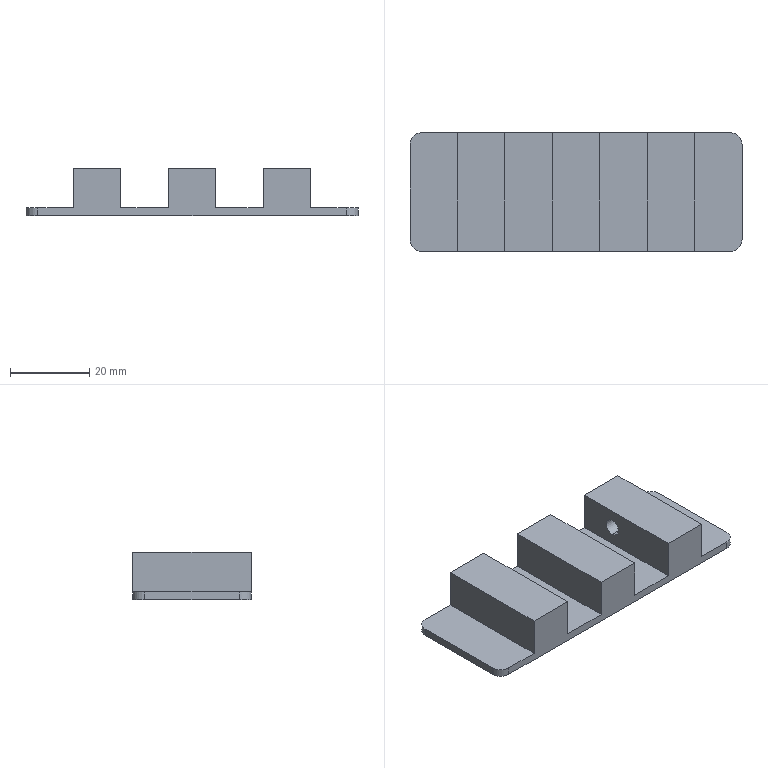Component | SolidWorks | SecondGenerationFour-sidedLabelingFeedingAdjustmentBaffle-1 | 1 solid | 24 faces | box 84 x 30 x 12 mm | volume 15658 mm3 | plane 18 | cylinder 6 | commonest cylinder face diameters 6 x4 4.2 x2
build123d program:
from build123d import *

# Parameters (mm, degrees)
SKETCH1_W             = 84
SKETCH1_H             = 30
BOSS_EXTRUDE1_DEPTH   = 6
SKETCH2_W             = 20
SKETCH2_H             = 53.944
SKETCH2_W_2           = 12
SKETCH2_H_2           = 79.849
SKETCH2_W_3           = 22.276
SKETCH2_H_3           = 76.76
CUT_EXTRUDE1_DEPTH    = 10
M5_TAPPED_HOLE1_D     = 4.2
M5_TAPPED_HOLE1_DEPTH = 19
M5_TAPPED_HOLE1_TIP   = 1.262
FILLET1_R             = 3


with BuildPart() as part:
    # Sketch1 → Boss-Extrude1 (new, symmetric)
    with BuildSketch(Plane.XY):
        Rectangle(SKETCH1_W, SKETCH1_H)
    extrude(amount=BOSS_EXTRUDE1_DEPTH, both=True)

    # Sketch2 → Cut-Extrude1 (cut)
    with BuildSketch(Plane.XY.offset(6)):
        with Locations((40, -0.6636)):
            Rectangle(SKETCH2_W, SKETCH2_H)
        with Locations((12, -0.6636)):
            Rectangle(SKETCH2_W_2, SKETCH2_H)
        with Locations((-12, 2.902)):
            Rectangle(SKETCH2_W_2, SKETCH2_H_2)
        with Locations((-41.138, 15.701)):
            Rectangle(SKETCH2_W_3, SKETCH2_H_3)
    extrude(amount=-CUT_EXTRUDE1_DEPTH, mode=Mode.SUBTRACT)

    # M5 Tapped Hole1
    with Locations(Plane(origin=(30, 0, 0), x_dir=(0, 0, -1), z_dir=(1, 0, 0))):
        with Locations((-1, 5)):
            Hole(M5_TAPPED_HOLE1_D / 2, depth=M5_TAPPED_HOLE1_DEPTH)
            with Locations((0, 0, -(M5_TAPPED_HOLE1_DEPTH + M5_TAPPED_HOLE1_TIP / 2))):  # 118° drill point
                Cone(0, M5_TAPPED_HOLE1_D / 2, M5_TAPPED_HOLE1_TIP, mode=Mode.SUBTRACT)

    # Fillet1
    fillet1_edges = [part.edges().sort_by_distance(p)[0] for p in [
        (42, -15, -5),
        (42, 15, -5),
        (-42, -15, -5),
        (-42, 15, -5),
    ]]
    fillet(fillet1_edges, radius=FILLET1_R)


solid = part.part

# Placed as in the assembly
solid = solid.moved(Location((9.973, 64.131, -120), (0, 0, 0)))
STEP:
#1=CARTESIAN_POINT('',(1.101,2.722,-4.602));
#2=VERTEX_POINT('',#1);
#3=CARTESIAN_POINT('',(1.101,2.722,-4.768));
#4=VERTEX_POINT('',#3);
#5=CARTESIAN_POINT('',(1.101,2.722,-4.685));
#6=DIRECTION('',(1.,0.,0.));
#7=DIRECTION('',(0.,1.,0.));
#8=AXIS2_PLACEMENT_3D('',#5,#6,#7);
#9=CIRCLE('',#8,0.08268);
#10=EDGE_CURVE('',#2,#4,#9,.T.);
#11=ORIENTED_EDGE('',*,*,#10,.F.);
#12=CARTESIAN_POINT('',(1.574,2.722,-4.602));
#13=VERTEX_POINT('',#12);
#14=CARTESIAN_POINT('',(1.574,2.722,-4.602));
#15=DIRECTION('',(1.,0.,0.));
#16=VECTOR('',#15,39.37);
#17=LINE('',#14,#16);
#18=EDGE_CURVE('',#2,#13,#17,.T.);
#19=ORIENTED_EDGE('',*,*,#18,.T.);
#20=CARTESIAN_POINT('',(1.574,2.722,-4.768));
#21=VERTEX_POINT('',#20);
#22=CARTESIAN_POINT('',(1.574,2.722,-4.685));
#23=DIRECTION('',(1.,0.,0.));
#24=DIRECTION('',(0.,0.,-1.));
#25=AXIS2_PLACEMENT_3D('',#22,#23,#24);
#26=CIRCLE('',#25,0.08268);
#27=EDGE_CURVE('',#13,#21,#26,.T.);
#28=ORIENTED_EDGE('',*,*,#27,.T.);
#29=CARTESIAN_POINT('',(1.574,2.722,-4.768));
#30=DIRECTION('',(1.,0.,0.));
#31=VECTOR('',#30,39.37);
#32=LINE('',#29,#31);
#33=EDGE_CURVE('',#4,#21,#32,.T.);
#34=ORIENTED_EDGE('',*,*,#33,.F.);
#35=EDGE_LOOP('',(#11,#19,#28,#34));
#36=FACE_OUTER_BOUND('',#35,.T.);
#37=CARTESIAN_POINT('',(1.574,2.722,-4.685));
#38=DIRECTION('',(1.,0.,0.));
#39=DIRECTION('',(0.,0.,-1.));
#40=AXIS2_PLACEMENT_3D('',#37,#38,#39);
#41=CYLINDRICAL_SURFACE('',#40,0.08268);
#42=ADVANCED_FACE('',(#36),#41,.F.);
#43=CARTESIAN_POINT('',(-1.261,2.997,-4.961));
#44=VERTEX_POINT('',#43);
#45=CARTESIAN_POINT('',(-1.261,2.052,-4.961));
#46=VERTEX_POINT('',#45);
#47=CARTESIAN_POINT('',(-1.261,1.934,-4.961));
#48=DIRECTION('',(0.,-1.,0.));
#49=VECTOR('',#48,39.37);
#50=LINE('',#47,#49);
#51=EDGE_CURVE('',#44,#46,#50,.T.);
#52=ORIENTED_EDGE('',*,*,#51,.T.);
#53=CARTESIAN_POINT('',(-1.261,2.052,-4.882));
#54=VERTEX_POINT('',#53);
#55=CARTESIAN_POINT('',(-1.261,2.052,-4.488));
#56=DIRECTION('',(0.,0.,1.));
#57=VECTOR('',#56,39.37);
#58=LINE('',#55,#57);
#59=EDGE_CURVE('',#46,#54,#58,.T.);
#60=ORIENTED_EDGE('',*,*,#59,.T.);
#61=CARTESIAN_POINT('',(-1.261,2.997,-4.882));
#62=VERTEX_POINT('',#61);
#63=CARTESIAN_POINT('',(-1.261,1.934,-4.882));
#64=DIRECTION('',(0.,-1.,0.));
#65=VECTOR('',#64,39.37);
#66=LINE('',#63,#65);
#67=EDGE_CURVE('',#62,#54,#66,.T.);
#68=ORIENTED_EDGE('',*,*,#67,.F.);
#69=CARTESIAN_POINT('',(-1.261,2.997,-4.488));
#70=DIRECTION('',(0.,0.,-1.));
#71=VECTOR('',#70,39.37);
#72=LINE('',#69,#71);
#73=EDGE_CURVE('',#62,#44,#72,.T.);
#74=ORIENTED_EDGE('',*,*,#73,.T.);
#75=EDGE_LOOP('',(#52,#60,#68,#74));
#76=FACE_OUTER_BOUND('',#75,.T.);
#77=CARTESIAN_POINT('',(-1.261,1.934,-4.488));
#78=DIRECTION('',(1.,0.,0.));
#79=DIRECTION('',(0.,0.,-1.));
#80=AXIS2_PLACEMENT_3D('',#77,#78,#79);
#81=PLANE('',#80);
#82=ADVANCED_FACE('',(#76),#81,.F.);
#83=CARTESIAN_POINT('',(-0.316,3.115,-4.488));
#84=VERTEX_POINT('',#83);
#85=CARTESIAN_POINT('',(-0.7885,3.115,-4.488));
#86=VERTEX_POINT('',#85);
#87=CARTESIAN_POINT('',(-1.261,3.115,-4.488));
#88=DIRECTION('',(-1.,0.,0.));
#89=VECTOR('',#88,39.37);
#90=LINE('',#87,#89);
#91=EDGE_CURVE('',#84,#86,#90,.T.);
#92=ORIENTED_EDGE('',*,*,#91,.T.);
#93=CARTESIAN_POINT('',(-0.7885,1.934,-4.488));
#94=VERTEX_POINT('',#93);
#95=CARTESIAN_POINT('',(-0.7885,4.654,-4.488));
#96=DIRECTION('',(-0.,1.,0.));
#97=VECTOR('',#96,39.37);
#98=LINE('',#95,#97);
#99=EDGE_CURVE('',#94,#86,#98,.T.);
#100=ORIENTED_EDGE('',*,*,#99,.F.);
#101=CARTESIAN_POINT('',(-0.316,1.934,-4.488));
#102=VERTEX_POINT('',#101);
#103=CARTESIAN_POINT('',(-1.261,1.934,-4.488));
#104=DIRECTION('',(1.,0.,0.));
#105=VECTOR('',#104,39.37);
#106=LINE('',#103,#105);
#107=EDGE_CURVE('',#94,#102,#106,.T.);
#108=ORIENTED_EDGE('',*,*,#107,.T.);
#109=CARTESIAN_POINT('',(-0.316,4.211,-4.488));
#110=DIRECTION('',(0.,-1.,0.));
#111=VECTOR('',#110,39.37);
#112=LINE('',#109,#111);
#113=EDGE_CURVE('',#84,#102,#112,.T.);
#114=ORIENTED_EDGE('',*,*,#113,.F.);
#115=EDGE_LOOP('',(#92,#100,#108,#114));
#116=FACE_OUTER_BOUND('',#115,.T.);
#117=CARTESIAN_POINT('',(2.046,3.115,-4.488));
#118=DIRECTION('',(0.,0.,-1.));
#119=DIRECTION('',(-1.,0.,0.));
#120=AXIS2_PLACEMENT_3D('',#117,#118,#119);
#121=PLANE('',#120);
#122=ADVANCED_FACE('',(#116),#121,.F.);
#123=CARTESIAN_POINT('',(0.6289,3.115,-4.488));
#124=VERTEX_POINT('',#123);
#125=CARTESIAN_POINT('',(0.1564,3.115,-4.488));
#126=VERTEX_POINT('',#125);
#127=CARTESIAN_POINT('',(-1.261,3.115,-4.488));
#128=DIRECTION('',(-1.,0.,0.));
#129=VECTOR('',#128,39.37);
#130=LINE('',#127,#129);
#131=EDGE_CURVE('',#124,#126,#130,.T.);
#132=ORIENTED_EDGE('',*,*,#131,.T.);
#133=CARTESIAN_POINT('',(0.1564,1.934,-4.488));
#134=VERTEX_POINT('',#133);
#135=CARTESIAN_POINT('',(0.1564,4.211,-4.488));
#136=DIRECTION('',(-0.,1.,0.));
#137=VECTOR('',#136,39.37);
#138=LINE('',#135,#137);
#139=EDGE_CURVE('',#134,#126,#138,.T.);
#140=ORIENTED_EDGE('',*,*,#139,.F.);
#141=CARTESIAN_POINT('',(0.6289,1.934,-4.488));
#142=VERTEX_POINT('',#141);
#143=CARTESIAN_POINT('',(-1.261,1.934,-4.488));
#144=DIRECTION('',(1.,0.,0.));
#145=VECTOR('',#144,39.37);
#146=LINE('',#143,#145);
#147=EDGE_CURVE('',#134,#142,#146,.T.);
#148=ORIENTED_EDGE('',*,*,#147,.T.);
#149=CARTESIAN_POINT('',(0.6289,3.115,-4.488));
#150=DIRECTION('',(-0.,1.,0.));
#151=VECTOR('',#150,39.37);
#152=LINE('',#149,#151);
#153=EDGE_CURVE('',#142,#124,#152,.T.);
#154=ORIENTED_EDGE('',*,*,#153,.T.);
#155=EDGE_LOOP('',(#132,#140,#148,#154));
#156=FACE_OUTER_BOUND('',#155,.T.);
#157=CARTESIAN_POINT('',(2.046,3.115,-4.488));
#158=DIRECTION('',(0.,0.,-1.));
#159=DIRECTION('',(-1.,0.,0.));
#160=AXIS2_PLACEMENT_3D('',#157,#158,#159);
#161=PLANE('',#160);
#162=ADVANCED_FACE('',(#156),#161,.F.);
#163=CARTESIAN_POINT('',(2.046,2.052,-4.882));
#164=VERTEX_POINT('',#163);
#165=CARTESIAN_POINT('',(2.046,2.997,-4.882));
#166=VERTEX_POINT('',#165);
#167=CARTESIAN_POINT('',(2.046,1.934,-4.882));
#168=DIRECTION('',(0.,1.,0.));
#169=VECTOR('',#168,39.37);
#170=LINE('',#167,#169);
#171=EDGE_CURVE('',#164,#166,#170,.T.);
#172=ORIENTED_EDGE('',*,*,#171,.F.);
#173=CARTESIAN_POINT('',(2.046,2.052,-4.961));
#174=VERTEX_POINT('',#173);
#175=CARTESIAN_POINT('',(2.046,2.052,-4.488));
#176=DIRECTION('',(0.,0.,-1.));
#177=VECTOR('',#176,39.37);
#178=LINE('',#175,#177);
#179=EDGE_CURVE('',#164,#174,#178,.T.);
#180=ORIENTED_EDGE('',*,*,#179,.T.);
#181=CARTESIAN_POINT('',(2.046,2.997,-4.961));
#182=VERTEX_POINT('',#181);
#183=CARTESIAN_POINT('',(2.046,1.934,-4.961));
#184=DIRECTION('',(0.,1.,0.));
#185=VECTOR('',#184,39.37);
#186=LINE('',#183,#185);
#187=EDGE_CURVE('',#174,#182,#186,.T.);
#188=ORIENTED_EDGE('',*,*,#187,.T.);
#189=CARTESIAN_POINT('',(2.046,2.997,-4.488));
#190=DIRECTION('',(0.,0.,1.));
#191=VECTOR('',#190,39.37);
#192=LINE('',#189,#191);
#193=EDGE_CURVE('',#182,#166,#192,.T.);
#194=ORIENTED_EDGE('',*,*,#193,.T.);
#195=EDGE_LOOP('',(#172,#180,#188,#194));
#196=FACE_OUTER_BOUND('',#195,.T.);
#197=CARTESIAN_POINT('',(2.046,1.934,-4.488));
#198=DIRECTION('',(-1.,0.,0.));
#199=DIRECTION('',(0.,0.,1.));
#200=AXIS2_PLACEMENT_3D('',#197,#198,#199);
#201=PLANE('',#200);
#202=ADVANCED_FACE('',(#196),#201,.F.);
#203=CARTESIAN_POINT('',(1.928,3.115,-4.961));
#204=VERTEX_POINT('',#203);
#205=CARTESIAN_POINT('',(-1.143,3.115,-4.961));
#206=VERTEX_POINT('',#205);
#207=CARTESIAN_POINT('',(-1.261,3.115,-4.961));
#208=DIRECTION('',(-1.,0.,0.));
#209=VECTOR('',#208,39.37);
#210=LINE('',#207,#209);
#211=EDGE_CURVE('',#204,#206,#210,.T.);
#212=ORIENTED_EDGE('',*,*,#211,.T.);
#213=CARTESIAN_POINT('',(-1.143,3.115,-4.882));
#214=VERTEX_POINT('',#213);
#215=CARTESIAN_POINT('',(-1.143,3.115,-4.488));
#216=DIRECTION('',(0.,0.,1.));
#217=VECTOR('',#216,39.37);
#218=LINE('',#215,#217);
#219=EDGE_CURVE('',#206,#214,#218,.T.);
#220=ORIENTED_EDGE('',*,*,#219,.T.);
#221=CARTESIAN_POINT('',(-0.7885,3.115,-4.882));
#222=VERTEX_POINT('',#221);
#223=CARTESIAN_POINT('',(-1.261,3.115,-4.882));
#224=DIRECTION('',(-1.,0.,0.));
#225=VECTOR('',#224,39.37);
#226=LINE('',#223,#225);
#227=EDGE_CURVE('',#222,#214,#226,.T.);
#228=ORIENTED_EDGE('',*,*,#227,.F.);
#229=CARTESIAN_POINT('',(-0.7885,3.115,-4.488));
#230=DIRECTION('',(0.,0.,1.));
#231=VECTOR('',#230,39.37);
#232=LINE('',#229,#231);
#233=EDGE_CURVE('',#222,#86,#232,.T.);
#234=ORIENTED_EDGE('',*,*,#233,.T.);
#235=ORIENTED_EDGE('',*,*,#91,.F.);
#236=CARTESIAN_POINT('',(-0.316,3.115,-4.882));
#237=VERTEX_POINT('',#236);
#238=CARTESIAN_POINT('',(-0.316,3.115,-4.488));
#239=DIRECTION('',(0.,0.,-1.));
#240=VECTOR('',#239,39.37);
#241=LINE('',#238,#240);
#242=EDGE_CURVE('',#84,#237,#241,.T.);
#243=ORIENTED_EDGE('',*,*,#242,.T.);
#244=CARTESIAN_POINT('',(0.1564,3.115,-4.882));
#245=VERTEX_POINT('',#244);
#246=CARTESIAN_POINT('',(-1.261,3.115,-4.882));
#247=DIRECTION('',(-1.,0.,0.));
#248=VECTOR('',#247,39.37);
#249=LINE('',#246,#248);
#250=EDGE_CURVE('',#245,#237,#249,.T.);
#251=ORIENTED_EDGE('',*,*,#250,.F.);
#252=CARTESIAN_POINT('',(0.1564,3.115,-4.488));
#253=DIRECTION('',(0.,0.,1.));
#254=VECTOR('',#253,39.37);
#255=LINE('',#252,#254);
#256=EDGE_CURVE('',#245,#126,#255,.T.);
#257=ORIENTED_EDGE('',*,*,#256,.T.);
#258=ORIENTED_EDGE('',*,*,#131,.F.);
#259=CARTESIAN_POINT('',(0.6289,3.115,-4.882));
#260=VERTEX_POINT('',#259);
#261=CARTESIAN_POINT('',(0.6289,3.115,-4.488));
#262=DIRECTION('',(0.,0.,-1.));
#263=VECTOR('',#262,39.37);
#264=LINE('',#261,#263);
#265=EDGE_CURVE('',#124,#260,#264,.T.);
#266=ORIENTED_EDGE('',*,*,#265,.T.);
#267=CARTESIAN_POINT('',(1.101,3.115,-4.882));
#268=VERTEX_POINT('',#267);
#269=CARTESIAN_POINT('',(-1.261,3.115,-4.882));
#270=DIRECTION('',(-1.,0.,0.));
#271=VECTOR('',#270,39.37);
#272=LINE('',#269,#271);
#273=EDGE_CURVE('',#268,#260,#272,.T.);
#274=ORIENTED_EDGE('',*,*,#273,.F.);
#275=CARTESIAN_POINT('',(1.101,3.115,-4.488));
#276=VERTEX_POINT('',#275);
#277=CARTESIAN_POINT('',(1.101,3.115,-4.488));
#278=DIRECTION('',(0.,0.,1.));
#279=VECTOR('',#278,39.37);
#280=LINE('',#277,#279);
#281=EDGE_CURVE('',#268,#276,#280,.T.);
#282=ORIENTED_EDGE('',*,*,#281,.T.);
#283=CARTESIAN_POINT('',(1.574,3.115,-4.488));
#284=VERTEX_POINT('',#283);
#285=CARTESIAN_POINT('',(-1.261,3.115,-4.488));
#286=DIRECTION('',(-1.,0.,0.));
#287=VECTOR('',#286,39.37);
#288=LINE('',#285,#287);
#289=EDGE_CURVE('',#284,#276,#288,.T.);
#290=ORIENTED_EDGE('',*,*,#289,.F.);
#291=CARTESIAN_POINT('',(1.574,3.115,-4.882));
#292=VERTEX_POINT('',#291);
#293=CARTESIAN_POINT('',(1.574,3.115,-4.488));
#294=DIRECTION('',(0.,0.,-1.));
#295=VECTOR('',#294,39.37);
#296=LINE('',#293,#295);
#297=EDGE_CURVE('',#284,#292,#296,.T.);
#298=ORIENTED_EDGE('',*,*,#297,.T.);
#299=CARTESIAN_POINT('',(1.928,3.115,-4.882));
#300=VERTEX_POINT('',#299);
#301=CARTESIAN_POINT('',(-1.261,3.115,-4.882));
#302=DIRECTION('',(-1.,0.,0.));
#303=VECTOR('',#302,39.37);
#304=LINE('',#301,#303);
#305=EDGE_CURVE('',#300,#292,#304,.T.);
#306=ORIENTED_EDGE('',*,*,#305,.F.);
#307=CARTESIAN_POINT('',(1.928,3.115,-4.488));
#308=DIRECTION('',(0.,0.,-1.));
#309=VECTOR('',#308,39.37);
#310=LINE('',#307,#309);
#311=EDGE_CURVE('',#300,#204,#310,.T.);
#312=ORIENTED_EDGE('',*,*,#311,.T.);
#313=EDGE_LOOP('',(#212,#220,#228,#234,#235,#243,#251,#257,#258,#266,#274,#282,#290,#298,#306,#312));
#314=FACE_OUTER_BOUND('',#313,.T.);
#315=CARTESIAN_POINT('',(-1.261,3.115,-4.488));
#316=DIRECTION('',(0.,-1.,0.));
#317=DIRECTION('',(0.,0.,-1.));
#318=AXIS2_PLACEMENT_3D('',#315,#316,#317);
#319=PLANE('',#318);
#320=ADVANCED_FACE('',(#314),#319,.F.);
#321=CARTESIAN_POINT('',(-1.143,1.934,-4.882));
#322=VERTEX_POINT('',#321);
#323=CARTESIAN_POINT('',(-0.7885,1.934,-4.882));
#324=VERTEX_POINT('',#323);
#325=CARTESIAN_POINT('',(-1.261,1.934,-4.882));
#326=DIRECTION('',(1.,0.,0.));
#327=VECTOR('',#326,39.37);
#328=LINE('',#325,#327);
#329=EDGE_CURVE('',#322,#324,#328,.T.);
#330=ORIENTED_EDGE('',*,*,#329,.F.);
#331=CARTESIAN_POINT('',(-1.143,1.934,-4.961));
#332=VERTEX_POINT('',#331);
#333=CARTESIAN_POINT('',(-1.143,1.934,-4.488));
#334=DIRECTION('',(0.,0.,-1.));
#335=VECTOR('',#334,39.37);
#336=LINE('',#333,#335);
#337=EDGE_CURVE('',#322,#332,#336,.T.);
#338=ORIENTED_EDGE('',*,*,#337,.T.);
#339=CARTESIAN_POINT('',(1.928,1.934,-4.961));
#340=VERTEX_POINT('',#339);
#341=CARTESIAN_POINT('',(-1.261,1.934,-4.961));
#342=DIRECTION('',(1.,0.,0.));
#343=VECTOR('',#342,39.37);
#344=LINE('',#341,#343);
#345=EDGE_CURVE('',#332,#340,#344,.T.);
#346=ORIENTED_EDGE('',*,*,#345,.T.);
#347=CARTESIAN_POINT('',(1.928,1.934,-4.882));
#348=VERTEX_POINT('',#347);
#349=CARTESIAN_POINT('',(1.928,1.934,-4.488));
#350=DIRECTION('',(0.,0.,1.));
#351=VECTOR('',#350,39.37);
#352=LINE('',#349,#351);
#353=EDGE_CURVE('',#340,#348,#352,.T.);
#354=ORIENTED_EDGE('',*,*,#353,.T.);
#355=CARTESIAN_POINT('',(1.574,1.934,-4.882));
#356=VERTEX_POINT('',#355);
#357=CARTESIAN_POINT('',(-1.261,1.934,-4.882));
#358=DIRECTION('',(1.,0.,0.));
#359=VECTOR('',#358,39.37);
#360=LINE('',#357,#359);
#361=EDGE_CURVE('',#356,#348,#360,.T.);
#362=ORIENTED_EDGE('',*,*,#361,.F.);
#363=CARTESIAN_POINT('',(1.574,1.934,-4.488));
#364=VERTEX_POINT('',#363);
#365=CARTESIAN_POINT('',(1.574,1.934,-4.488));
#366=DIRECTION('',(0.,0.,1.));
#367=VECTOR('',#366,39.37);
#368=LINE('',#365,#367);
#369=EDGE_CURVE('',#356,#364,#368,.T.);
#370=ORIENTED_EDGE('',*,*,#369,.T.);
#371=CARTESIAN_POINT('',(1.101,1.934,-4.488));
#372=VERTEX_POINT('',#371);
#373=CARTESIAN_POINT('',(-1.261,1.934,-4.488));
#374=DIRECTION('',(1.,0.,0.));
#375=VECTOR('',#374,39.37);
#376=LINE('',#373,#375);
#377=EDGE_CURVE('',#372,#364,#376,.T.);
#378=ORIENTED_EDGE('',*,*,#377,.F.);
#379=CARTESIAN_POINT('',(1.101,1.934,-4.882));
#380=VERTEX_POINT('',#379);
#381=CARTESIAN_POINT('',(1.101,1.934,-4.488));
#382=DIRECTION('',(0.,0.,-1.));
#383=VECTOR('',#382,39.37);
#384=LINE('',#381,#383);
#385=EDGE_CURVE('',#372,#380,#384,.T.);
#386=ORIENTED_EDGE('',*,*,#385,.T.);
#387=CARTESIAN_POINT('',(0.6289,1.934,-4.882));
#388=VERTEX_POINT('',#387);
#389=CARTESIAN_POINT('',(-1.261,1.934,-4.882));
#390=DIRECTION('',(1.,0.,0.));
#391=VECTOR('',#390,39.37);
#392=LINE('',#389,#391);
#393=EDGE_CURVE('',#388,#380,#392,.T.);
#394=ORIENTED_EDGE('',*,*,#393,.F.);
#395=CARTESIAN_POINT('',(0.6289,1.934,-4.488));
#396=DIRECTION('',(0.,0.,1.));
#397=VECTOR('',#396,39.37);
#398=LINE('',#395,#397);
#399=EDGE_CURVE('',#388,#142,#398,.T.);
#400=ORIENTED_EDGE('',*,*,#399,.T.);
#401=ORIENTED_EDGE('',*,*,#147,.F.);
#402=CARTESIAN_POINT('',(0.1564,1.934,-4.882));
#403=VERTEX_POINT('',#402);
#404=CARTESIAN_POINT('',(0.1564,1.934,-4.488));
#405=DIRECTION('',(0.,0.,-1.));
#406=VECTOR('',#405,39.37);
#407=LINE('',#404,#406);
#408=EDGE_CURVE('',#134,#403,#407,.T.);
#409=ORIENTED_EDGE('',*,*,#408,.T.);
#410=CARTESIAN_POINT('',(-0.316,1.934,-4.882));
#411=VERTEX_POINT('',#410);
#412=CARTESIAN_POINT('',(-1.261,1.934,-4.882));
#413=DIRECTION('',(1.,0.,0.));
#414=VECTOR('',#413,39.37);
#415=LINE('',#412,#414);
#416=EDGE_CURVE('',#411,#403,#415,.T.);
#417=ORIENTED_EDGE('',*,*,#416,.F.);
#418=CARTESIAN_POINT('',(-0.316,1.934,-4.488));
#419=DIRECTION('',(0.,0.,1.));
#420=VECTOR('',#419,39.37);
#421=LINE('',#418,#420);
#422=EDGE_CURVE('',#411,#102,#421,.T.);
#423=ORIENTED_EDGE('',*,*,#422,.T.);
#424=ORIENTED_EDGE('',*,*,#107,.F.);
#425=CARTESIAN_POINT('',(-0.7885,1.934,-4.488));
#426=DIRECTION('',(0.,0.,-1.));
#427=VECTOR('',#426,39.37);
#428=LINE('',#425,#427);
#429=EDGE_CURVE('',#94,#324,#428,.T.);
#430=ORIENTED_EDGE('',*,*,#429,.T.);
#431=EDGE_LOOP('',(#330,#338,#346,#354,#362,#370,#378,#386,#394,#400,#401,#409,#417,#423,#424,#430));
#432=FACE_OUTER_BOUND('',#431,.T.);
#433=CARTESIAN_POINT('',(-1.261,1.934,-4.488));
#434=DIRECTION('',(0.,1.,0.));
#435=DIRECTION('',(0.,0.,1.));
#436=AXIS2_PLACEMENT_3D('',#433,#434,#435);
#437=PLANE('',#436);
#438=ADVANCED_FACE('',(#432),#437,.F.);
#439=ORIENTED_EDGE('',*,*,#289,.T.);
#440=CARTESIAN_POINT('',(1.101,3.115,-4.488));
#441=DIRECTION('',(0.,-1.,0.));
#442=VECTOR('',#441,39.37);
#443=LINE('',#440,#442);
#444=EDGE_CURVE('',#276,#372,#443,.T.);
#445=ORIENTED_EDGE('',*,*,#444,.T.);
#446=ORIENTED_EDGE('',*,*,#377,.T.);
#447=CARTESIAN_POINT('',(1.574,3.115,-4.488));
#448=DIRECTION('',(-0.,1.,0.));
#449=VECTOR('',#448,39.37);
#450=LINE('',#447,#449);
#451=EDGE_CURVE('',#364,#284,#450,.T.);
#452=ORIENTED_EDGE('',*,*,#451,.T.);
#453=EDGE_LOOP('',(#439,#445,#446,#452));
#454=FACE_OUTER_BOUND('',#453,.T.);
#455=CARTESIAN_POINT('',(2.046,3.115,-4.488));
#456=DIRECTION('',(0.,0.,-1.));
#457=DIRECTION('',(-1.,0.,0.));
#458=AXIS2_PLACEMENT_3D('',#455,#456,#457);
#459=PLANE('',#458);
#460=ADVANCED_FACE('',(#454),#459,.F.);
#461=ORIENTED_EDGE('',*,*,#345,.F.);
#462=CARTESIAN_POINT('',(-1.143,2.052,-4.961));
#463=DIRECTION('',(0.,0.,-1.));
#464=DIRECTION('',(-1.,0.,0.));
#465=AXIS2_PLACEMENT_3D('',#462,#463,#464);
#466=CIRCLE('',#465,0.1181);
#467=EDGE_CURVE('',#332,#46,#466,.T.);
#468=ORIENTED_EDGE('',*,*,#467,.T.);
#469=ORIENTED_EDGE('',*,*,#51,.F.);
#470=CARTESIAN_POINT('',(-1.143,2.997,-4.961));
#471=DIRECTION('',(0.,0.,-1.));
#472=DIRECTION('',(-1.,0.,0.));
#473=AXIS2_PLACEMENT_3D('',#470,#471,#472);
#474=CIRCLE('',#473,0.1181);
#475=EDGE_CURVE('',#44,#206,#474,.T.);
#476=ORIENTED_EDGE('',*,*,#475,.T.);
#477=ORIENTED_EDGE('',*,*,#211,.F.);
#478=CARTESIAN_POINT('',(1.928,2.997,-4.961));
#479=DIRECTION('',(0.,0.,-1.));
#480=DIRECTION('',(-1.,0.,0.));
#481=AXIS2_PLACEMENT_3D('',#478,#479,#480);
#482=CIRCLE('',#481,0.1181);
#483=EDGE_CURVE('',#204,#182,#482,.T.);
#484=ORIENTED_EDGE('',*,*,#483,.T.);
#485=ORIENTED_EDGE('',*,*,#187,.F.);
#486=CARTESIAN_POINT('',(1.928,2.052,-4.961));
#487=DIRECTION('',(0.,0.,-1.));
#488=DIRECTION('',(-1.,0.,0.));
#489=AXIS2_PLACEMENT_3D('',#486,#487,#488);
#490=CIRCLE('',#489,0.1181);
#491=EDGE_CURVE('',#174,#340,#490,.T.);
#492=ORIENTED_EDGE('',*,*,#491,.T.);
#493=EDGE_LOOP('',(#461,#468,#469,#476,#477,#484,#485,#492));
#494=FACE_OUTER_BOUND('',#493,.T.);
#495=CARTESIAN_POINT('',(2.046,3.115,-4.961));
#496=DIRECTION('',(0.,0.,-1.));
#497=DIRECTION('',(-1.,0.,0.));
#498=AXIS2_PLACEMENT_3D('',#495,#496,#497);
#499=PLANE('',#498);
#500=ADVANCED_FACE('',(#494),#499,.T.);
#501=ORIENTED_EDGE('',*,*,#361,.T.);
#502=CARTESIAN_POINT('',(1.928,2.052,-4.882));
#503=DIRECTION('',(0.,0.,1.));
#504=DIRECTION('',(1.,0.,0.));
#505=AXIS2_PLACEMENT_3D('',#502,#503,#504);
#506=CIRCLE('',#505,0.1181);
#507=EDGE_CURVE('',#348,#164,#506,.T.);
#508=ORIENTED_EDGE('',*,*,#507,.T.);
#509=ORIENTED_EDGE('',*,*,#171,.T.);
#510=CARTESIAN_POINT('',(1.928,2.997,-4.882));
#511=DIRECTION('',(0.,0.,1.));
#512=DIRECTION('',(1.,0.,0.));
#513=AXIS2_PLACEMENT_3D('',#510,#511,#512);
#514=CIRCLE('',#513,0.1181);
#515=EDGE_CURVE('',#166,#300,#514,.T.);
#516=ORIENTED_EDGE('',*,*,#515,.T.);
#517=ORIENTED_EDGE('',*,*,#305,.T.);
#518=CARTESIAN_POINT('',(1.574,3.561,-4.882));
#519=DIRECTION('',(0.,-1.,0.));
#520=VECTOR('',#519,39.37);
#521=LINE('',#518,#520);
#522=EDGE_CURVE('',#292,#356,#521,.T.);
#523=ORIENTED_EDGE('',*,*,#522,.T.);
#524=EDGE_LOOP('',(#501,#508,#509,#516,#517,#523));
#525=FACE_OUTER_BOUND('',#524,.T.);
#526=CARTESIAN_POINT('',(1.574,1.437,-4.882));
#527=DIRECTION('',(0.,0.,1.));
#528=DIRECTION('',(1.,0.,0.));
#529=AXIS2_PLACEMENT_3D('',#526,#527,#528);
#530=PLANE('',#529);
#531=ADVANCED_FACE('',(#525),#530,.T.);
#532=CARTESIAN_POINT('',(1.574,2.722,-4.685));
#533=DIRECTION('',(1.,0.,0.));
#534=DIRECTION('',(0.,0.,-1.));
#535=AXIS2_PLACEMENT_3D('',#532,#533,#534);
#536=CIRCLE('',#535,0.08268);
#537=EDGE_CURVE('',#21,#13,#536,.T.);
#538=ORIENTED_EDGE('',*,*,#537,.F.);
#539=ORIENTED_EDGE('',*,*,#27,.F.);
#540=EDGE_LOOP('',(#538,#539));
#541=FACE_BOUND('',#540,.T.);
#542=ORIENTED_EDGE('',*,*,#451,.F.);
#543=ORIENTED_EDGE('',*,*,#369,.F.);
#544=ORIENTED_EDGE('',*,*,#522,.F.);
#545=ORIENTED_EDGE('',*,*,#297,.F.);
#546=EDGE_LOOP('',(#542,#543,#544,#545));
#547=FACE_OUTER_BOUND('',#546,.T.);
#548=CARTESIAN_POINT('',(1.574,3.561,-4.882));
#549=DIRECTION('',(-1.,-0.,0.));
#550=DIRECTION('',(0.,-1.,0.));
#551=AXIS2_PLACEMENT_3D('',#548,#549,#550);
#552=PLANE('',#551);
#553=ADVANCED_FACE('',(#541,#547),#552,.F.);
#554=ORIENTED_EDGE('',*,*,#273,.T.);
#555=CARTESIAN_POINT('',(0.6289,3.561,-4.882));
#556=DIRECTION('',(0.,-1.,0.));
#557=VECTOR('',#556,39.37);
#558=LINE('',#555,#557);
#559=EDGE_CURVE('',#260,#388,#558,.T.);
#560=ORIENTED_EDGE('',*,*,#559,.T.);
#561=ORIENTED_EDGE('',*,*,#393,.T.);
#562=CARTESIAN_POINT('',(1.101,3.561,-4.882));
#563=DIRECTION('',(-0.,1.,0.));
#564=VECTOR('',#563,39.37);
#565=LINE('',#562,#564);
#566=EDGE_CURVE('',#380,#268,#565,.T.);
#567=ORIENTED_EDGE('',*,*,#566,.T.);
#568=EDGE_LOOP('',(#554,#560,#561,#567));
#569=FACE_OUTER_BOUND('',#568,.T.);
#570=CARTESIAN_POINT('',(0.6289,1.437,-4.882));
#571=DIRECTION('',(0.,0.,1.));
#572=DIRECTION('',(1.,0.,0.));
#573=AXIS2_PLACEMENT_3D('',#570,#571,#572);
#574=PLANE('',#573);
#575=ADVANCED_FACE('',(#569),#574,.T.);
#576=ORIENTED_EDGE('',*,*,#153,.F.);
#577=ORIENTED_EDGE('',*,*,#399,.F.);
#578=ORIENTED_EDGE('',*,*,#559,.F.);
#579=ORIENTED_EDGE('',*,*,#265,.F.);
#580=EDGE_LOOP('',(#576,#577,#578,#579));
#581=FACE_OUTER_BOUND('',#580,.T.);
#582=CARTESIAN_POINT('',(0.6289,3.561,-4.882));
#583=DIRECTION('',(-1.,-0.,0.));
#584=DIRECTION('',(0.,-1.,0.));
#585=AXIS2_PLACEMENT_3D('',#582,#583,#584);
#586=PLANE('',#585);
#587=ADVANCED_FACE('',(#581),#586,.F.);
#588=CARTESIAN_POINT('',(1.101,2.722,-4.685));
#589=DIRECTION('',(1.,0.,0.));
#590=DIRECTION('',(0.,1.,0.));
#591=AXIS2_PLACEMENT_3D('',#588,#589,#590);
#592=CIRCLE('',#591,0.08268);
#593=EDGE_CURVE('',#4,#2,#592,.T.);
#594=ORIENTED_EDGE('',*,*,#593,.T.);
#595=ORIENTED_EDGE('',*,*,#10,.T.);
#596=EDGE_LOOP('',(#594,#595));
#597=FACE_BOUND('',#596,.T.);
#598=ORIENTED_EDGE('',*,*,#566,.F.);
#599=ORIENTED_EDGE('',*,*,#385,.F.);
#600=ORIENTED_EDGE('',*,*,#444,.F.);
#601=ORIENTED_EDGE('',*,*,#281,.F.);
#602=EDGE_LOOP('',(#598,#599,#600,#601));
#603=FACE_OUTER_BOUND('',#602,.T.);
#604=CARTESIAN_POINT('',(1.101,3.561,-4.882));
#605=DIRECTION('',(1.,0.,0.));
#606=DIRECTION('',(-0.,1.,0.));
#607=AXIS2_PLACEMENT_3D('',#604,#605,#606);
#608=PLANE('',#607);
#609=ADVANCED_FACE('',(#597,#603),#608,.F.);
#610=ORIENTED_EDGE('',*,*,#113,.T.);
#611=ORIENTED_EDGE('',*,*,#422,.F.);
#612=CARTESIAN_POINT('',(-0.316,4.211,-4.882));
#613=DIRECTION('',(0.,-1.,0.));
#614=VECTOR('',#613,39.37);
#615=LINE('',#612,#614);
#616=EDGE_CURVE('',#237,#411,#615,.T.);
#617=ORIENTED_EDGE('',*,*,#616,.F.);
#618=ORIENTED_EDGE('',*,*,#242,.F.);
#619=EDGE_LOOP('',(#610,#611,#617,#618));
#620=FACE_OUTER_BOUND('',#619,.T.);
#621=CARTESIAN_POINT('',(-0.316,4.211,-4.882));
#622=DIRECTION('',(-1.,-0.,0.));
#623=DIRECTION('',(0.,-1.,0.));
#624=AXIS2_PLACEMENT_3D('',#621,#622,#623);
#625=PLANE('',#624);
#626=ADVANCED_FACE('',(#620),#625,.F.);
#627=CARTESIAN_POINT('',(0.1564,4.211,-4.882));
#628=DIRECTION('',(-0.,1.,0.));
#629=VECTOR('',#628,39.37);
#630=LINE('',#627,#629);
#631=EDGE_CURVE('',#403,#245,#630,.T.);
#632=ORIENTED_EDGE('',*,*,#631,.F.);
#633=ORIENTED_EDGE('',*,*,#408,.F.);
#634=ORIENTED_EDGE('',*,*,#139,.T.);
#635=ORIENTED_EDGE('',*,*,#256,.F.);
#636=EDGE_LOOP('',(#632,#633,#634,#635));
#637=FACE_OUTER_BOUND('',#636,.T.);
#638=CARTESIAN_POINT('',(0.1564,4.211,-4.882));
#639=DIRECTION('',(1.,0.,0.));
#640=DIRECTION('',(-0.,1.,0.));
#641=AXIS2_PLACEMENT_3D('',#638,#639,#640);
#642=PLANE('',#641);
#643=ADVANCED_FACE('',(#637),#642,.F.);
#644=ORIENTED_EDGE('',*,*,#250,.T.);
#645=ORIENTED_EDGE('',*,*,#616,.T.);
#646=ORIENTED_EDGE('',*,*,#416,.T.);
#647=ORIENTED_EDGE('',*,*,#631,.T.);
#648=EDGE_LOOP('',(#644,#645,#646,#647));
#649=FACE_OUTER_BOUND('',#648,.T.);
#650=CARTESIAN_POINT('',(-0.316,1.067,-4.882));
#651=DIRECTION('',(0.,0.,1.));
#652=DIRECTION('',(1.,0.,0.));
#653=AXIS2_PLACEMENT_3D('',#650,#651,#652);
#654=PLANE('',#653);
#655=ADVANCED_FACE('',(#649),#654,.T.);
#656=CARTESIAN_POINT('',(-0.7885,4.654,-4.882));
#657=DIRECTION('',(-0.,1.,0.));
#658=VECTOR('',#657,39.37);
#659=LINE('',#656,#658);
#660=EDGE_CURVE('',#324,#222,#659,.T.);
#661=ORIENTED_EDGE('',*,*,#660,.F.);
#662=ORIENTED_EDGE('',*,*,#429,.F.);
#663=ORIENTED_EDGE('',*,*,#99,.T.);
#664=ORIENTED_EDGE('',*,*,#233,.F.);
#665=EDGE_LOOP('',(#661,#662,#663,#664));
#666=FACE_OUTER_BOUND('',#665,.T.);
#667=CARTESIAN_POINT('',(-0.7885,4.654,-4.882));
#668=DIRECTION('',(1.,0.,0.));
#669=DIRECTION('',(-0.,1.,0.));
#670=AXIS2_PLACEMENT_3D('',#667,#668,#669);
#671=PLANE('',#670);
#672=ADVANCED_FACE('',(#666),#671,.F.);
#673=ORIENTED_EDGE('',*,*,#67,.T.);
#674=CARTESIAN_POINT('',(-1.143,2.052,-4.882));
#675=DIRECTION('',(0.,0.,1.));
#676=DIRECTION('',(1.,0.,0.));
#677=AXIS2_PLACEMENT_3D('',#674,#675,#676);
#678=CIRCLE('',#677,0.1181);
#679=EDGE_CURVE('',#54,#322,#678,.T.);
#680=ORIENTED_EDGE('',*,*,#679,.T.);
#681=ORIENTED_EDGE('',*,*,#329,.T.);
#682=ORIENTED_EDGE('',*,*,#660,.T.);
#683=ORIENTED_EDGE('',*,*,#227,.T.);
#684=CARTESIAN_POINT('',(-1.143,2.997,-4.882));
#685=DIRECTION('',(0.,0.,1.));
#686=DIRECTION('',(1.,0.,0.));
#687=AXIS2_PLACEMENT_3D('',#684,#685,#686);
#688=CIRCLE('',#687,0.1181);
#689=EDGE_CURVE('',#214,#62,#688,.T.);
#690=ORIENTED_EDGE('',*,*,#689,.T.);
#691=EDGE_LOOP('',(#673,#680,#681,#682,#683,#690));
#692=FACE_OUTER_BOUND('',#691,.T.);
#693=CARTESIAN_POINT('',(-1.665,1.632,-4.882));
#694=DIRECTION('',(0.,0.,1.));
#695=DIRECTION('',(1.,0.,0.));
#696=AXIS2_PLACEMENT_3D('',#693,#694,#695);
#697=PLANE('',#696);
#698=ADVANCED_FACE('',(#692),#697,.T.);
#699=ORIENTED_EDGE('',*,*,#18,.F.);
#700=ORIENTED_EDGE('',*,*,#593,.F.);
#701=ORIENTED_EDGE('',*,*,#33,.T.);
#702=ORIENTED_EDGE('',*,*,#537,.T.);
#703=EDGE_LOOP('',(#699,#700,#701,#702));
#704=FACE_OUTER_BOUND('',#703,.T.);
#705=CARTESIAN_POINT('',(1.574,2.722,-4.685));
#706=DIRECTION('',(1.,0.,0.));
#707=DIRECTION('',(0.,0.,-1.));
#708=AXIS2_PLACEMENT_3D('',#705,#706,#707);
#709=CYLINDRICAL_SURFACE('',#708,0.08268);
#710=ADVANCED_FACE('',(#704),#709,.F.);
#711=ORIENTED_EDGE('',*,*,#679,.F.);
#712=ORIENTED_EDGE('',*,*,#59,.F.);
#713=ORIENTED_EDGE('',*,*,#467,.F.);
#714=ORIENTED_EDGE('',*,*,#337,.F.);
#715=EDGE_LOOP('',(#711,#712,#713,#714));
#716=FACE_OUTER_BOUND('',#715,.T.);
#717=CARTESIAN_POINT('',(-1.143,2.052,-4.488));
#718=DIRECTION('',(0.,0.,-1.));
#719=DIRECTION('',(-1.,0.,0.));
#720=AXIS2_PLACEMENT_3D('',#717,#718,#719);
#721=CYLINDRICAL_SURFACE('',#720,0.1181);
#722=ADVANCED_FACE('',(#716),#721,.T.);
#723=ORIENTED_EDGE('',*,*,#689,.F.);
#724=ORIENTED_EDGE('',*,*,#219,.F.);
#725=ORIENTED_EDGE('',*,*,#475,.F.);
#726=ORIENTED_EDGE('',*,*,#73,.F.);
#727=EDGE_LOOP('',(#723,#724,#725,#726));
#728=FACE_OUTER_BOUND('',#727,.T.);
#729=CARTESIAN_POINT('',(-1.143,2.997,-4.488));
#730=DIRECTION('',(0.,0.,-1.));
#731=DIRECTION('',(-1.,0.,0.));
#732=AXIS2_PLACEMENT_3D('',#729,#730,#731);
#733=CYLINDRICAL_SURFACE('',#732,0.1181);
#734=ADVANCED_FACE('',(#728),#733,.T.);
#735=ORIENTED_EDGE('',*,*,#507,.F.);
#736=ORIENTED_EDGE('',*,*,#353,.F.);
#737=ORIENTED_EDGE('',*,*,#491,.F.);
#738=ORIENTED_EDGE('',*,*,#179,.F.);
#739=EDGE_LOOP('',(#735,#736,#737,#738));
#740=FACE_OUTER_BOUND('',#739,.T.);
#741=CARTESIAN_POINT('',(1.928,2.052,-4.488));
#742=DIRECTION('',(0.,0.,-1.));
#743=DIRECTION('',(-1.,0.,0.));
#744=AXIS2_PLACEMENT_3D('',#741,#742,#743);
#745=CYLINDRICAL_SURFACE('',#744,0.1181);
#746=ADVANCED_FACE('',(#740),#745,.T.);
#747=ORIENTED_EDGE('',*,*,#515,.F.);
#748=ORIENTED_EDGE('',*,*,#193,.F.);
#749=ORIENTED_EDGE('',*,*,#483,.F.);
#750=ORIENTED_EDGE('',*,*,#311,.F.);
#751=EDGE_LOOP('',(#747,#748,#749,#750));
#752=FACE_OUTER_BOUND('',#751,.T.);
#753=CARTESIAN_POINT('',(1.928,2.997,-4.488));
#754=DIRECTION('',(0.,0.,-1.));
#755=DIRECTION('',(-1.,0.,0.));
#756=AXIS2_PLACEMENT_3D('',#753,#754,#755);
#757=CYLINDRICAL_SURFACE('',#756,0.1181);
#758=ADVANCED_FACE('',(#752),#757,.T.);
#759=CLOSED_SHELL('',(#42,#82,#122,#162,#202,#320,#438,#460,#500,#531,#553,#575,#587,#609,#626,#643,#655,#672,#698,#710,#722,#734,#746,#758));
#760=MANIFOLD_SOLID_BREP('',#759);
#761=CARTESIAN_POINT('',(0.,0.,0.));
#762=DIRECTION('',(0.,0.,1.));
#763=DIRECTION('',(1.,0.,0.));
#764=AXIS2_PLACEMENT_3D('',#761,#762,#763);
#765=(LENGTH_UNIT()NAMED_UNIT(*)SI_UNIT($,.METRE.));
#766=LENGTH_MEASURE_WITH_UNIT(LENGTH_MEASURE(0.0254),#765);
#767=DIMENSIONAL_EXPONENTS(1.,0.,0.,0.,0.,0.,0.);
#768=(CONVERSION_BASED_UNIT('',#766)LENGTH_UNIT()NAMED_UNIT(#767));
#769=UNCERTAINTY_MEASURE_WITH_UNIT(LENGTH_MEASURE(0.00001),#768,'','');
#770=(NAMED_UNIT(*)PLANE_ANGLE_UNIT()SI_UNIT($,.RADIAN.));
#771=(NAMED_UNIT(*)SI_UNIT($,.STERADIAN.)SOLID_ANGLE_UNIT());
#772=(GEOMETRIC_REPRESENTATION_CONTEXT(3)GLOBAL_UNCERTAINTY_ASSIGNED_CONTEXT((#769))GLOBAL_UNIT_ASSIGNED_CONTEXT((#768,#770,#771))REPRESENTATION_CONTEXT('',''));
#773=ADVANCED_BREP_SHAPE_REPRESENTATION('',(#760,#764),#772);
#774=COLOUR_RGB('',0.7922,0.8196,0.9333);
#775=FILL_AREA_STYLE_COLOUR('',#774);
#776=FILL_AREA_STYLE('',(#775));
#777=SURFACE_STYLE_FILL_AREA(#776);
#778=SURFACE_SIDE_STYLE('',(#777));
#779=SURFACE_STYLE_USAGE(.BOTH.,#778);
#780=PRESENTATION_STYLE_ASSIGNMENT((#779));
#781=STYLED_ITEM('',(#780),#760);
#782=PRESENTATION_LAYER_ASSIGNMENT('','',(#781));
#783=(LENGTH_UNIT()NAMED_UNIT(*)SI_UNIT($,.METRE.));
#784=LENGTH_MEASURE_WITH_UNIT(LENGTH_MEASURE(0.0254),#783);
#785=DIMENSIONAL_EXPONENTS(1.,0.,0.,0.,0.,0.,0.);
#786=(CONVERSION_BASED_UNIT('',#784)LENGTH_UNIT()NAMED_UNIT(#785));
#787=UNCERTAINTY_MEASURE_WITH_UNIT(LENGTH_MEASURE(0.00001),#786,'','');
#788=(NAMED_UNIT(*)PLANE_ANGLE_UNIT()SI_UNIT($,.RADIAN.));
#789=(NAMED_UNIT(*)SI_UNIT($,.STERADIAN.)SOLID_ANGLE_UNIT());
#790=(GEOMETRIC_REPRESENTATION_CONTEXT(3)GLOBAL_UNCERTAINTY_ASSIGNED_CONTEXT((#787))GLOBAL_UNIT_ASSIGNED_CONTEXT((#786,#788,#789))REPRESENTATION_CONTEXT('',''));
#791=MECHANICAL_DESIGN_GEOMETRIC_PRESENTATION_REPRESENTATION('',(#781),#790);